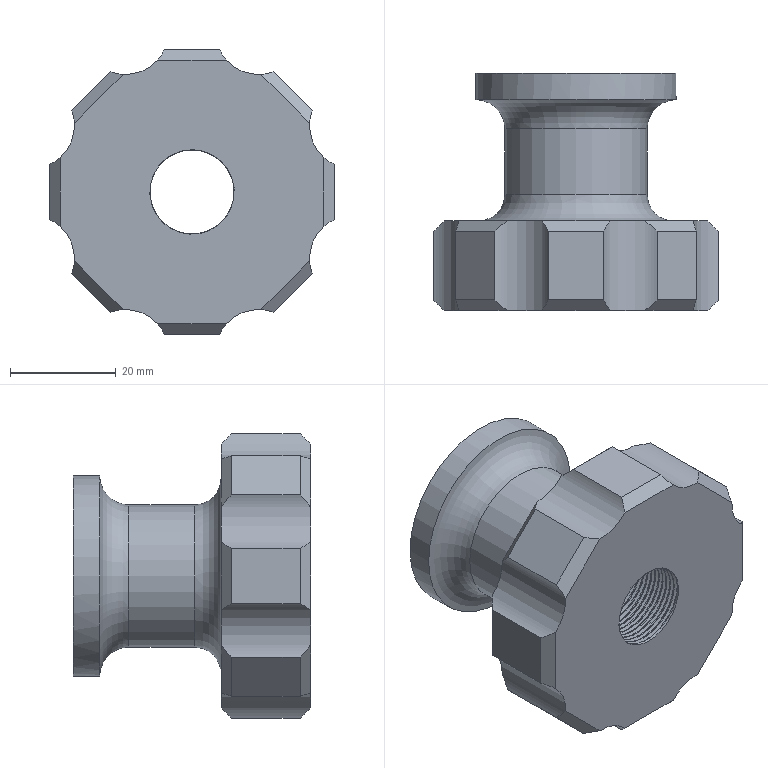Component | NX | HAND_NUT | 1 solid | 44 faces | volume 47461 mm3 | plane 28 | cylinder 12 | torus 2 | spline 2 | commonest cylinder face diameters 16 x9 27 x1 38 x1 17 x1